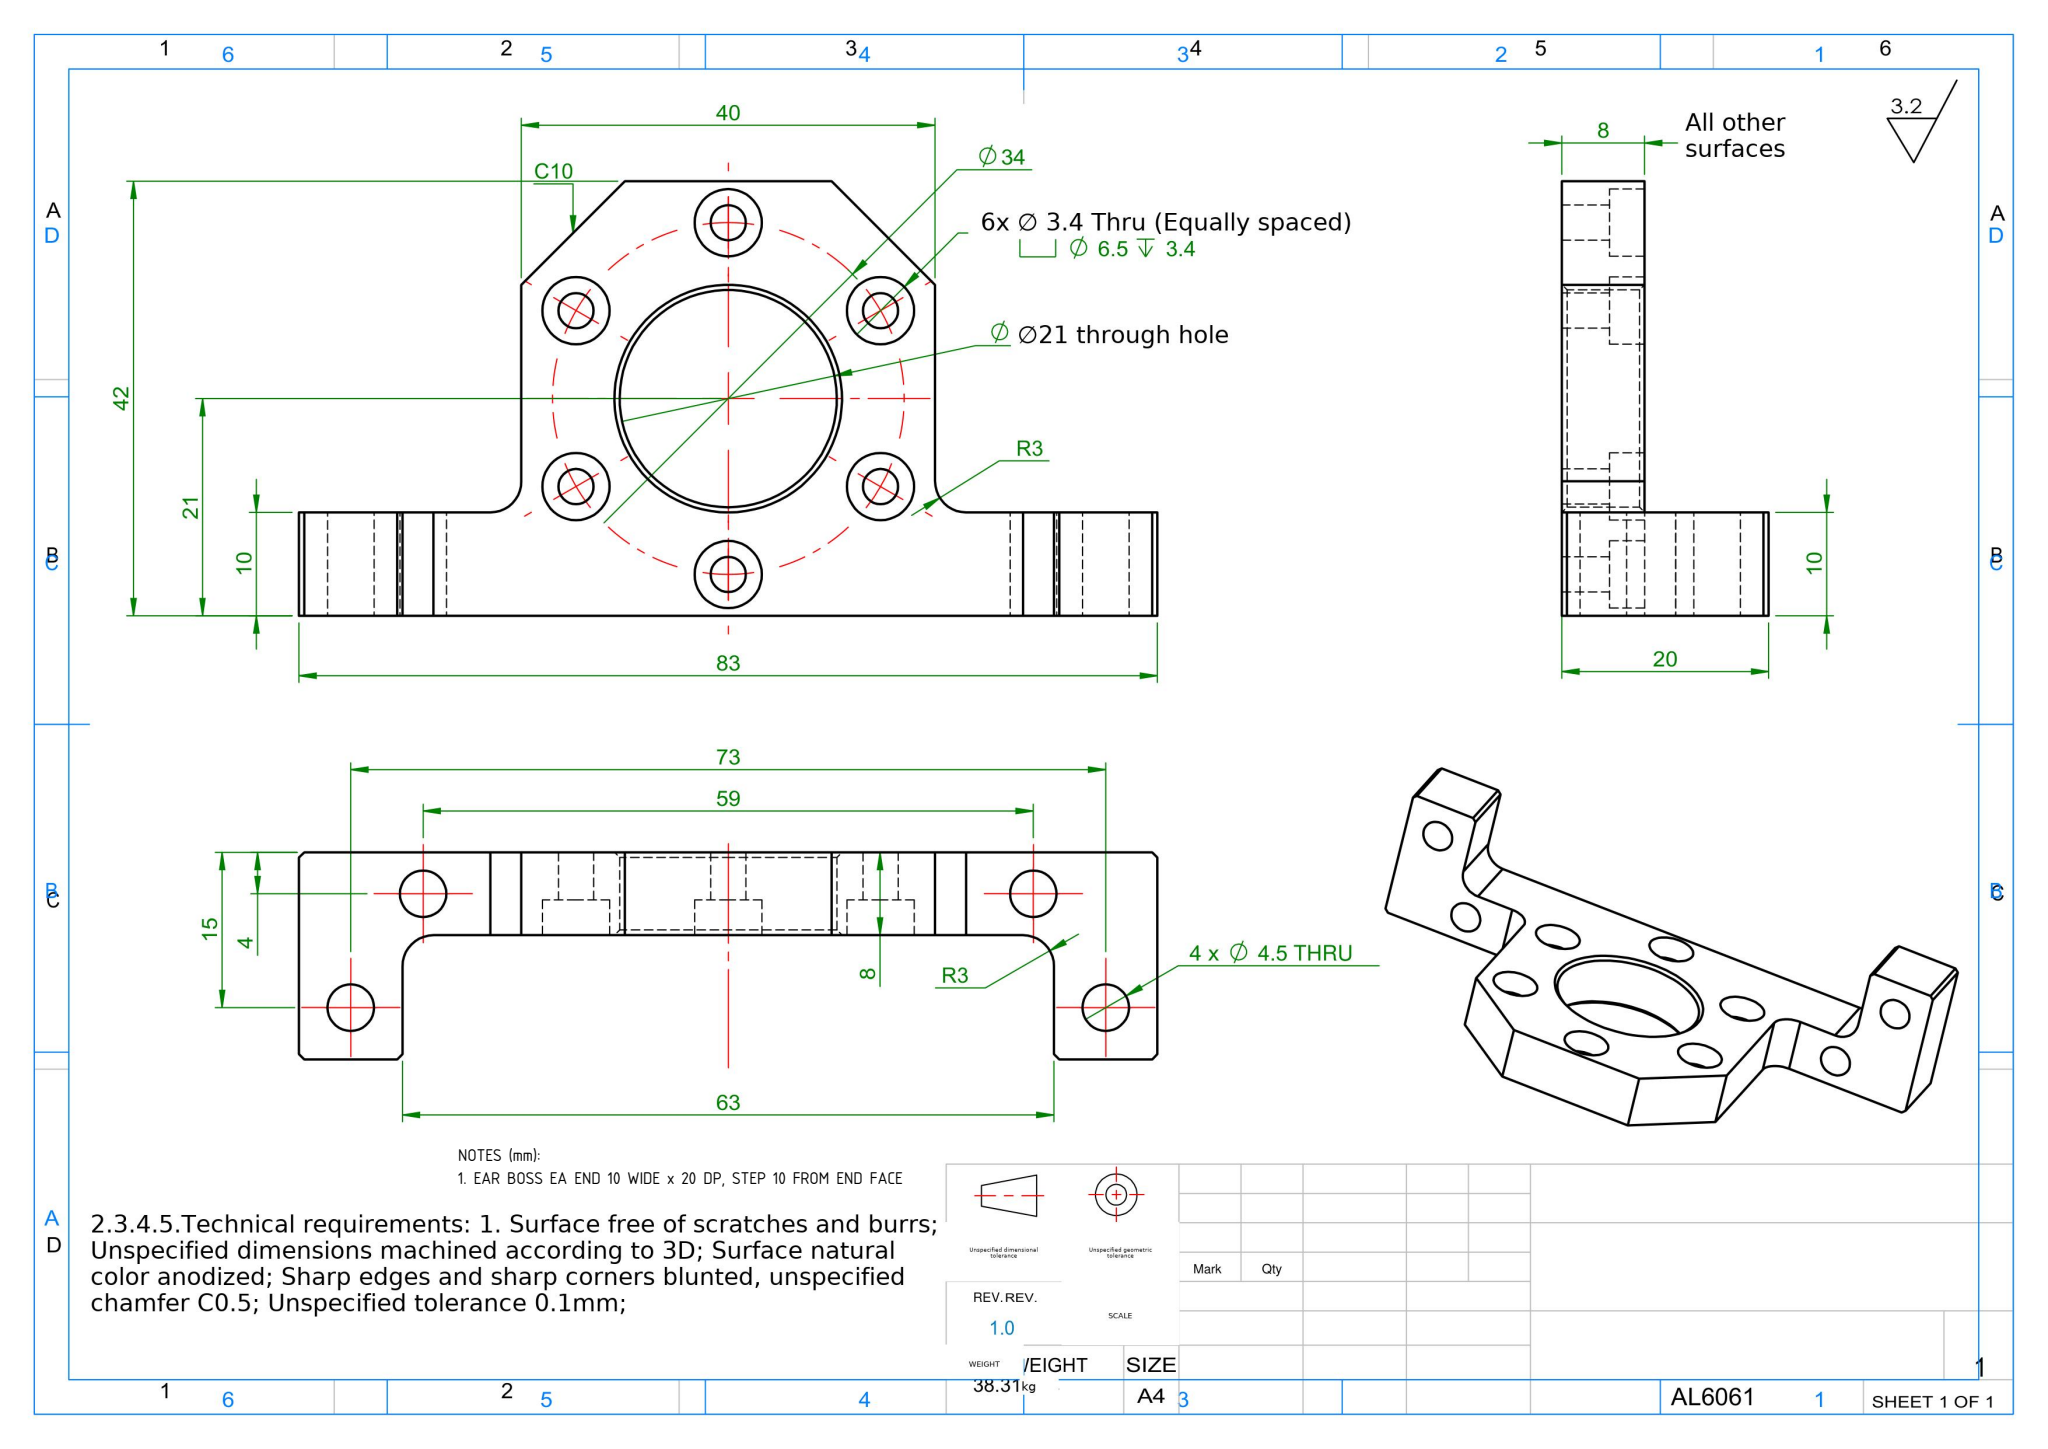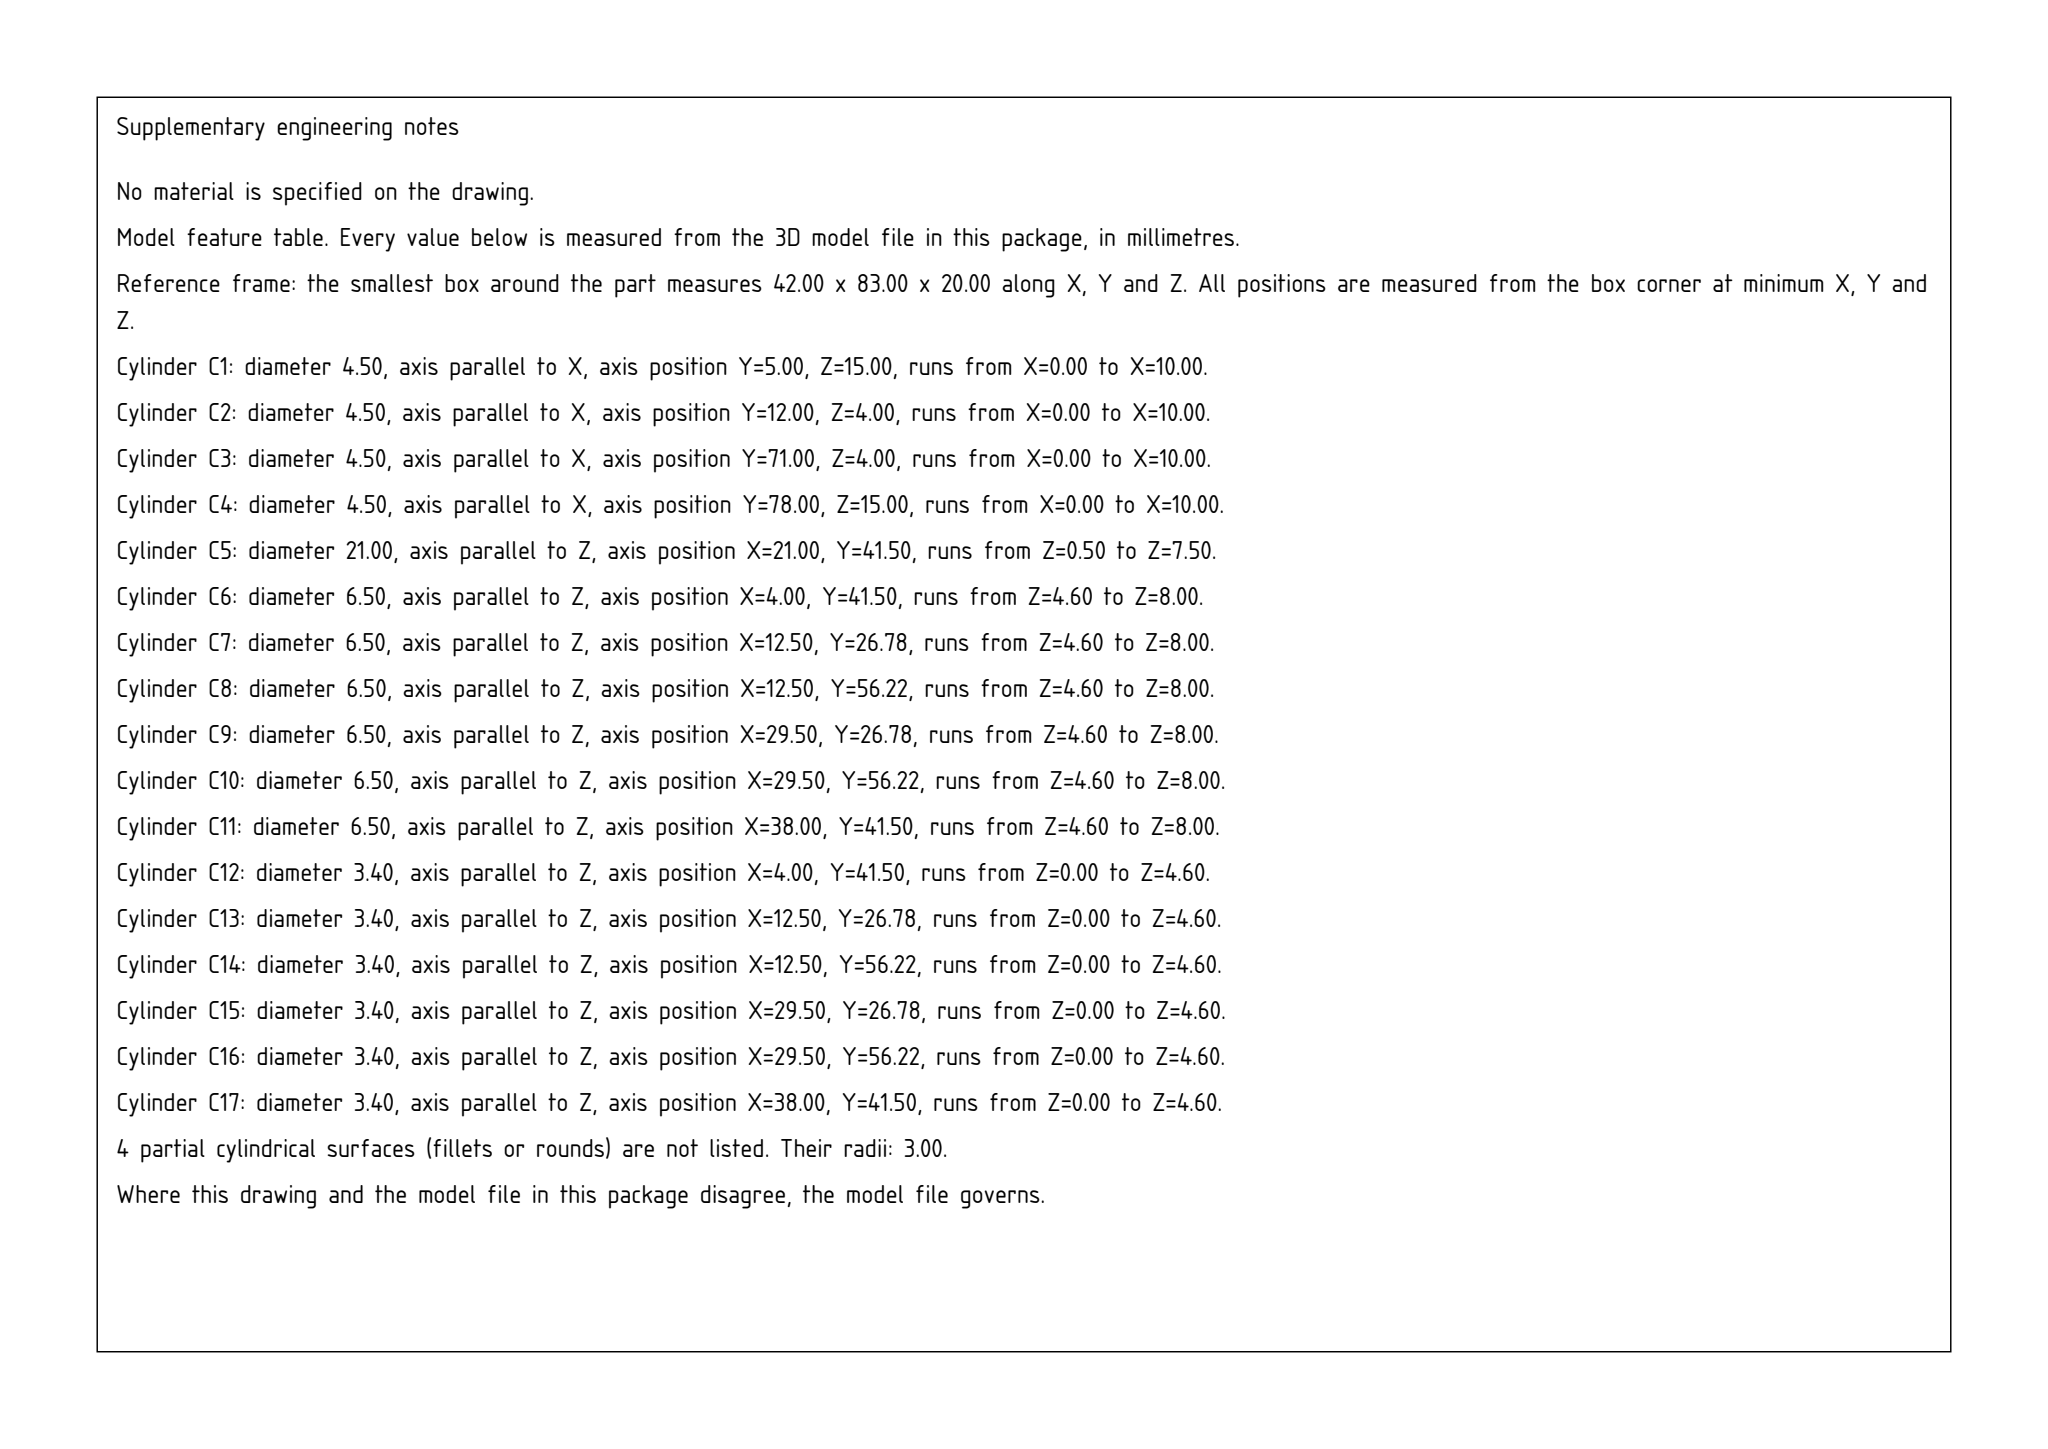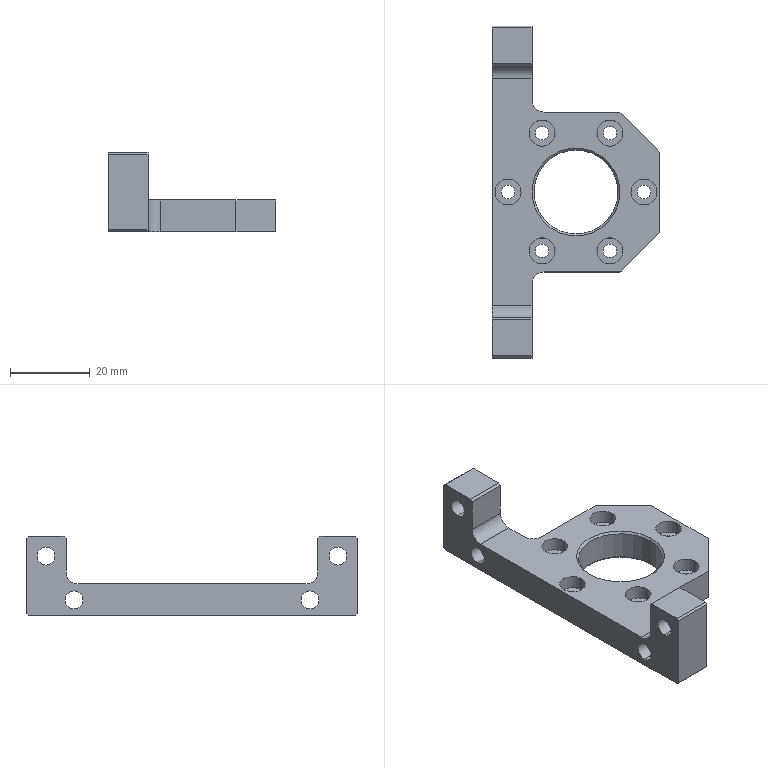Part | SolidWorks | mm | 1 solid | 70 faces | box 42 x 83 x 20 mm | volume 14191 mm3 | cylinder 38 | plane 28 | cone 4 | commonest cylinder face diameters 6.5 x12 3.4 x12 4.5 x8 6 x4 21 x2
Drawing notes:
EAR BOSS EA END 10 WIDE x 20 DP, STEP 10 FROM END FACE | from the solid: Ear top faces z=20 over x 0-10, y 0.5-9.5 and y 73.5-82.5 (10 wide, top at z=20, 10 deep in x); ear step faces are planes y=10 and y=73 (x 0-10, z 11-19.5), i.e. 10 from each end face (y=0 / y=83), blended by R3 fillets (dia 6, axis x) at y=13/70, z=11. The 21.5 planes (x 13-32, z 0-8) belong to the octagonal plate, not the ear.
build123d program:
from build123d import *

# Parameters (mm, degrees)
SKETCH1_R                                       = 20
SKETCH1_R_2                                     = 10.5
BOSS_EXTRUDE1_DEPTH                             = 6
SKETCH4_W                                       = 42
SKETCH4_H                                       = 83
SKETCH4_R                                       = 10.5
BOSS_EXTRUDE2_DEPTH                             = 20
SKETCH8_W                                       = 42
SKETCH8_H                                       = 63
CUT_EXTRUDE2_DEPTH                              = 12
M3_HEX_SOCKET_HEAD_CAP_SCREW_CBORE1_D           = 3.4
M3_HEX_SOCKET_HEAD_CAP_SCREW_CBORE1_CBORE_D     = 6.5
M3_HEX_SOCKET_HEAD_CAP_SCREW_CBORE1_CBORE_DEPTH = 3.4
CIRPATTERN1_COUNT                               = 6
SKETCH17_W                                      = 32
SKETCH17_H                                      = 83
CUT_EXTRUDE4_DEPTH                              = 49.034
SKETCH18_W                                      = 32
SKETCH18_H                                      = 21.5
CUT_EXTRUDE5_DEPTH                              = 49.034
FILLET2_R                                       = 3
M4_CLEARANCE_HOLE1_D                            = 4.5
CHAMFER1_SIZE                                   = 10
CHAMFER2_SIZE                                   = 0.5


with BuildPart() as part:
    # Sketch1 → Boss-Extrude1 (new body)
    with BuildSketch(Plane.XY):
        Circle(SKETCH1_R)
        Circle(SKETCH1_R_2, mode=Mode.SUBTRACT)
    extrude(amount=BOSS_EXTRUDE1_DEPTH)

    # Sketch4 → Boss-Extrude2 (add)
    with BuildSketch(Plane(origin=(0, 0, 0), x_dir=(-1, 0, 0), z_dir=(0, 0, -1))):
        Rectangle(SKETCH4_W, SKETCH4_H)
        Circle(SKETCH4_R, mode=Mode.SUBTRACT)
    extrude(amount=-BOSS_EXTRUDE2_DEPTH)

    # Sketch8 → Cut-Extrude2 (cut)
    with BuildSketch(Plane.XY.offset(20)):
        Rectangle(SKETCH8_W, SKETCH8_H)
    extrude(amount=-CUT_EXTRUDE2_DEPTH, mode=Mode.SUBTRACT)

    # M3 Hex Socket Head Cap Screw CBORE1 (through all)
    with Locations(Plane.XY.offset(8)):
        with Locations((-17, 0)):
            m3_hex_socket_head_cap_screw_cbore1 = CounterBoreHole(M3_HEX_SOCKET_HEAD_CAP_SCREW_CBORE1_D / 2, M3_HEX_SOCKET_HEAD_CAP_SCREW_CBORE1_CBORE_D / 2, M3_HEX_SOCKET_HEAD_CAP_SCREW_CBORE1_CBORE_DEPTH)

    # CirPattern1: M3 Hex Socket Head Cap Screw CBORE1 ×6 about axis
    cirpattern1_axis = Axis((0, 0, 0), (0, 0, 1))
    for i in range(1, CIRPATTERN1_COUNT):
        add(m3_hex_socket_head_cap_screw_cbore1.rotate(cirpattern1_axis, i * 360 / CIRPATTERN1_COUNT), mode=Mode.SUBTRACT)

    # Sketch17 → Cut-Extrude4 (cut, through all)
    with BuildSketch(Plane.XY.offset(8)):
        with Locations((5, 0)):
            Rectangle(SKETCH17_W, SKETCH17_H)
    extrude(amount=CUT_EXTRUDE4_DEPTH, mode=Mode.SUBTRACT)

    # Sketch18 → Cut-Extrude5 (cut, through all)
    with BuildSketch(Plane.XY.offset(8)):
        with Locations((5, -30.75)):
            Rectangle(SKETCH18_W, SKETCH18_H)
        with Locations((5, 30.75)):
            Rectangle(SKETCH18_W, SKETCH18_H)
    extrude(amount=-CUT_EXTRUDE5_DEPTH, mode=Mode.SUBTRACT)

    # Fillet2
    fillet2_edges = [part.edges().sort_by_distance(p)[0] for p in [
        (-11, -20, 4),
        (-11, 20, 4),
        (-16, -31.5, 8),
        (-16, 31.5, 8),
    ]]
    fillet(fillet2_edges, radius=FILLET2_R)

    # M4 Clearance Hole1 (through all)
    with Locations(Plane(origin=(-11, 0, 0), x_dir=(0, 0, -1), z_dir=(1, 0, 0))):
        with Locations((-15, 36.5), (-4, 29.5), (-4, -29.5), (-15, -36.5)):
            Hole(M4_CLEARANCE_HOLE1_D / 2)

    # Chamfer1
    chamfer1_edges = [part.edges().sort_by_distance(p)[0] for p in [
        (21, -20, 4),
        (21, 20, 4),
    ]]
    chamfer(chamfer1_edges, length=CHAMFER1_SIZE)

    # Chamfer2
    chamfer2_edges = [part.edges().sort_by_distance(p)[0] for p in [
        (-16, 41.5, 0),
        (-16, 41.5, 20),
        (-16, -41.5, 0),
        (10.5, 0, 8),
        (-16, -31.5, 20),
        (0, -10.5, 0),
        (-16, 31.5, 20),
        (-16, -41.5, 20),
    ]]
    chamfer(chamfer2_edges, length=CHAMFER2_SIZE)


solid = part.part